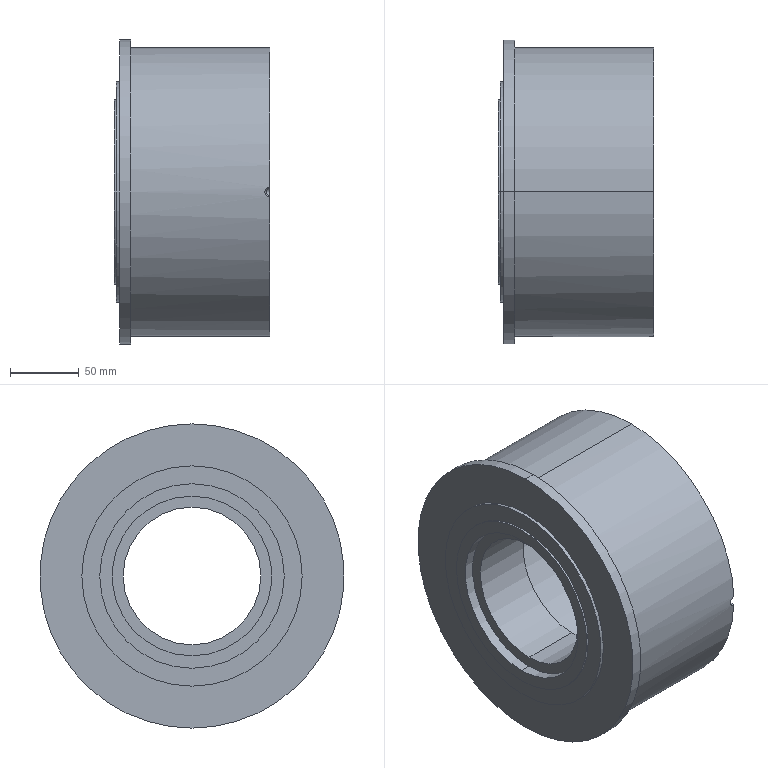Component | SolidWorks | PistonCylinder-1 | 1 solid | 54 faces | volume 2082765 mm3 | cylinder 33 | plane 13 | cone 8 | commonest cylinder face diameters 5 x9 6 x6 3 x2 116 x2 134 x2 160 x2 221 x2 210 x2